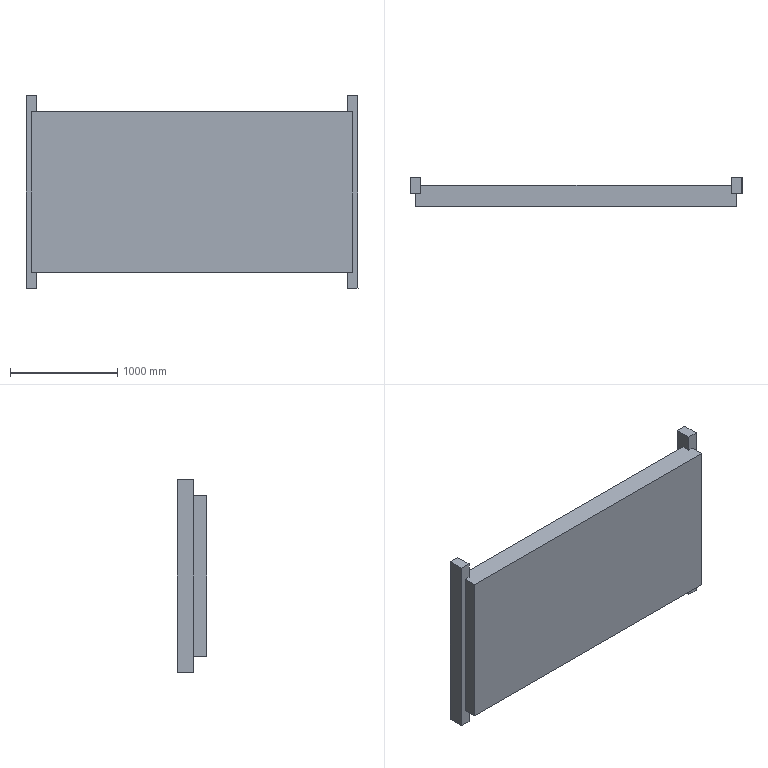Component | SolidWorks | LiftingAndOperatingMechanism-1_21-1 | 1 solid | 18 faces | box 3100 x 275 x 1800 mm | volume 942750000 mm3 | plane 18
build123d program:
from build123d import *

# Parameters (mm, degrees)
SKETCH2_W           = 500
SKETCH2_H           = 800
SKETCH2_W_2         = 440
SKETCH2_H_2         = 740
EXTRUDE_THIN1_DEPTH = 300
SKETCH3_W           = 440
SKETCH3_H           = 240
CUT_EXTRUDE1_DEPTH  = 8353.85
SKETCH4_W           = 740
SKETCH4_H           = 240
CUT_EXTRUDE2_DEPTH  = 8325.662
SKETCH5_W           = 1500
SKETCH5_H           = 3000
BOSS_EXTRUDE1_DEPTH = 100
SKETCH6_W           = 1800
SKETCH6_H           = 150
BOSS_EXTRUDE2_DEPTH = 50
SKETCH9_W           = 1500
SKETCH9_H           = 3000
CUT_EXTRUDE3_DEPTH  = 1944.637


with BuildPart() as part:
    # Sketch2 → Extrude-Thin1 (new body)
    with BuildSketch(Plane(origin=(0, -8000, 0), x_dir=(1, 0, 0), z_dir=(0, 1, 0))):
        with Locations((240, 0)):
            Rectangle(SKETCH2_W, SKETCH2_H)
        with Locations((240, 0)):
            Rectangle(SKETCH2_W_2, SKETCH2_H_2, mode=Mode.SUBTRACT)
    extrude(amount=-EXTRUDE_THIN1_DEPTH)

    # Sketch3 → Cut-Extrude1 (cut, through all)
    with BuildSketch(Plane.XY.offset(400)):
        with Locations((240, -8150)):
            Rectangle(SKETCH3_W, SKETCH3_H)
    extrude(amount=-CUT_EXTRUDE1_DEPTH, mode=Mode.SUBTRACT)

    # Sketch4 → Cut-Extrude2 (cut, through all)
    with BuildSketch(Plane(origin=(490, 0, 0), x_dir=(0, 0, -1), z_dir=(1, 0, 0))):
        with Locations((0, -8150)):
            Rectangle(SKETCH4_W, SKETCH4_H)
    extrude(amount=-CUT_EXTRUDE2_DEPTH, mode=Mode.SUBTRACT)

    # Sketch5 → Boss-Extrude1 (add, symmetric)
    with BuildSketch(Plane.XZ.offset(8300)):
        with Locations((240, 0)):
            Rectangle(SKETCH5_W, SKETCH5_H)
    extrude(amount=BOSS_EXTRUDE1_DEPTH, both=True)

    # Sketch6 → Boss-Extrude2 (add, symmetric)
    with BuildSketch(Plane.XY.offset(1500)):
        with Locations((240, -8400)):
            Rectangle(SKETCH6_W, SKETCH6_H)
    boss_extrude2 = extrude(amount=BOSS_EXTRUDE2_DEPTH, both=True)

    # Mirror1: Boss-Extrude2 across plane
    add(boss_extrude2.mirror(Plane.XY))

    # Sketch9 → Cut-Extrude3 (cut, through all)
    with BuildSketch(Plane(origin=(0, -8200, 0), x_dir=(1, 0, 0), z_dir=(0, 1, 0))):
        with Locations((240, 0)):
            Rectangle(SKETCH9_W, SKETCH9_H)
    extrude(amount=CUT_EXTRUDE3_DEPTH, mode=Mode.SUBTRACT)


solid = part.part

# Placed as in the assembly
solid = solid.moved(Location((-258.963, 11809.183, 6107.842), (180, 90, 0)))
STEP:
#1=COLOUR_RGB('',0.7922,0.8196,0.9333);
#2=FILL_AREA_STYLE_COLOUR('',#1);
#3=FILL_AREA_STYLE('',(#2));
#4=SURFACE_STYLE_FILL_AREA(#3);
#5=SURFACE_SIDE_STYLE('',(#4));
#6=SURFACE_STYLE_USAGE(.BOTH.,#5);
#7=PRESENTATION_STYLE_ASSIGNMENT((#6));
#8=CARTESIAN_POINT('',(46.891,795.637,220.388));
#9=VERTEX_POINT('',#8);
#10=CARTESIAN_POINT('',(-67.282,795.637,220.387));
#11=VERTEX_POINT('',#10);
#12=CARTESIAN_POINT('',(48.86,795.637,220.388));
#13=DIRECTION('',(-1.,-0.,-0.00000094));
#14=VECTOR('',#13,39.37);
#15=LINE('',#12,#14);
#16=EDGE_CURVE('',#9,#11,#15,.T.);
#17=ORIENTED_EDGE('',*,*,#16,.T.);
#18=CARTESIAN_POINT('',(-67.282,795.637,279.443));
#19=VERTEX_POINT('',#18);
#20=CARTESIAN_POINT('',(-67.282,795.637,240.466));
#21=DIRECTION('',(-0.00000094,-0.,1.));
#22=VECTOR('',#21,39.37);
#23=LINE('',#20,#22);
#24=EDGE_CURVE('',#11,#19,#23,.T.);
#25=ORIENTED_EDGE('',*,*,#24,.T.);
#26=CARTESIAN_POINT('',(46.891,795.637,279.443));
#27=VERTEX_POINT('',#26);
#28=CARTESIAN_POINT('',(48.86,795.637,279.443));
#29=DIRECTION('',(1.,0.,0.00000094));
#30=VECTOR('',#29,39.37);
#31=LINE('',#28,#30);
#32=EDGE_CURVE('',#19,#27,#31,.T.);
#33=ORIENTED_EDGE('',*,*,#32,.T.);
#34=CARTESIAN_POINT('',(46.891,795.637,240.466));
#35=DIRECTION('',(0.00000094,0.,-1.));
#36=VECTOR('',#35,39.37);
#37=LINE('',#34,#36);
#38=EDGE_CURVE('',#27,#9,#37,.T.);
#39=ORIENTED_EDGE('',*,*,#38,.T.);
#40=EDGE_LOOP('',(#17,#25,#33,#39));
#41=FACE_OUTER_BOUND('',#40,.T.);
#42=CARTESIAN_POINT('',(-10.195,795.637,240.466));
#43=DIRECTION('',(-0.,1.,0.));
#44=DIRECTION('',(-1.,-0.,-0.00000094));
#45=AXIS2_PLACEMENT_3D('',#42,#43,#44);
#46=PLANE('',#45);
#47=ADVANCED_FACE('',(#41),#46,.T.);
#48=CARTESIAN_POINT('',(-67.282,792.684,279.443));
#49=VERTEX_POINT('',#48);
#50=CARTESIAN_POINT('',(-67.282,795.637,279.443));
#51=DIRECTION('',(-0.,1.,0.));
#52=VECTOR('',#51,39.37);
#53=LINE('',#50,#52);
#54=EDGE_CURVE('',#49,#19,#53,.T.);
#55=ORIENTED_EDGE('',*,*,#54,.F.);
#56=CARTESIAN_POINT('',(-69.251,792.684,279.443));
#57=VERTEX_POINT('',#56);
#58=CARTESIAN_POINT('',(48.86,792.684,279.443));
#59=DIRECTION('',(-1.,-0.,-0.00000094));
#60=VECTOR('',#59,39.37);
#61=LINE('',#58,#60);
#62=EDGE_CURVE('',#49,#57,#61,.T.);
#63=ORIENTED_EDGE('',*,*,#62,.T.);
#64=CARTESIAN_POINT('',(-69.251,787.763,279.443));
#65=VERTEX_POINT('',#64);
#66=CARTESIAN_POINT('',(-69.251,795.637,279.443));
#67=DIRECTION('',(0.,-1.,-0.));
#68=VECTOR('',#67,39.37);
#69=LINE('',#66,#68);
#70=EDGE_CURVE('',#57,#65,#69,.T.);
#71=ORIENTED_EDGE('',*,*,#70,.T.);
#72=CARTESIAN_POINT('',(48.86,787.763,279.443));
#73=VERTEX_POINT('',#72);
#74=CARTESIAN_POINT('',(48.86,787.763,279.443));
#75=DIRECTION('',(1.,0.,0.00000094));
#76=VECTOR('',#75,39.37);
#77=LINE('',#74,#76);
#78=EDGE_CURVE('',#65,#73,#77,.T.);
#79=ORIENTED_EDGE('',*,*,#78,.T.);
#80=CARTESIAN_POINT('',(48.86,792.684,279.443));
#81=VERTEX_POINT('',#80);
#82=CARTESIAN_POINT('',(48.86,795.637,279.443));
#83=DIRECTION('',(0.,-1.,-0.));
#84=VECTOR('',#83,39.37);
#85=LINE('',#82,#84);
#86=EDGE_CURVE('',#81,#73,#85,.T.);
#87=ORIENTED_EDGE('',*,*,#86,.F.);
#88=CARTESIAN_POINT('',(46.891,792.684,279.443));
#89=VERTEX_POINT('',#88);
#90=CARTESIAN_POINT('',(48.86,792.684,279.443));
#91=DIRECTION('',(1.,0.,0.00000094));
#92=VECTOR('',#91,39.37);
#93=LINE('',#90,#92);
#94=EDGE_CURVE('',#89,#81,#93,.T.);
#95=ORIENTED_EDGE('',*,*,#94,.F.);
#96=CARTESIAN_POINT('',(46.891,795.637,279.443));
#97=DIRECTION('',(0.,-1.,-0.));
#98=VECTOR('',#97,39.37);
#99=LINE('',#96,#98);
#100=EDGE_CURVE('',#27,#89,#99,.T.);
#101=ORIENTED_EDGE('',*,*,#100,.F.);
#102=ORIENTED_EDGE('',*,*,#32,.F.);
#103=EDGE_LOOP('',(#55,#63,#71,#79,#87,#95,#101,#102));
#104=FACE_OUTER_BOUND('',#103,.T.);
#105=CARTESIAN_POINT('',(48.86,795.637,279.443));
#106=DIRECTION('',(0.00000094,0.,-1.));
#107=DIRECTION('',(1.,0.,0.00000094));
#108=AXIS2_PLACEMENT_3D('',#105,#106,#107);
#109=PLANE('',#108);
#110=ADVANCED_FACE('',(#104),#109,.F.);
#111=CARTESIAN_POINT('',(48.86,792.684,220.388));
#112=VERTEX_POINT('',#111);
#113=CARTESIAN_POINT('',(48.86,792.684,220.388));
#114=DIRECTION('',(0.00000094,0.,-1.));
#115=VECTOR('',#114,39.37);
#116=LINE('',#113,#115);
#117=EDGE_CURVE('',#81,#112,#116,.T.);
#118=ORIENTED_EDGE('',*,*,#117,.F.);
#119=ORIENTED_EDGE('',*,*,#86,.T.);
#120=CARTESIAN_POINT('',(48.86,787.763,220.388));
#121=VERTEX_POINT('',#120);
#122=CARTESIAN_POINT('',(48.86,787.763,220.388));
#123=DIRECTION('',(0.00000094,0.,-1.));
#124=VECTOR('',#123,39.37);
#125=LINE('',#122,#124);
#126=EDGE_CURVE('',#73,#121,#125,.T.);
#127=ORIENTED_EDGE('',*,*,#126,.T.);
#128=CARTESIAN_POINT('',(48.86,795.637,220.388));
#129=DIRECTION('',(0.,-1.,-0.));
#130=VECTOR('',#129,39.37);
#131=LINE('',#128,#130);
#132=EDGE_CURVE('',#112,#121,#131,.T.);
#133=ORIENTED_EDGE('',*,*,#132,.F.);
#134=EDGE_LOOP('',(#118,#119,#127,#133));
#135=FACE_OUTER_BOUND('',#134,.T.);
#136=CARTESIAN_POINT('',(48.86,795.637,220.388));
#137=DIRECTION('',(-1.,-0.,-0.00000094));
#138=DIRECTION('',(0.00000094,0.,-1.));
#139=AXIS2_PLACEMENT_3D('',#136,#137,#138);
#140=PLANE('',#139);
#141=ADVANCED_FACE('',(#135),#140,.F.);
#142=CARTESIAN_POINT('',(-69.25,792.684,220.387));
#143=VERTEX_POINT('',#142);
#144=CARTESIAN_POINT('',(-69.25,787.763,220.387));
#145=VERTEX_POINT('',#144);
#146=CARTESIAN_POINT('',(-69.25,795.637,220.387));
#147=DIRECTION('',(0.,-1.,-0.));
#148=VECTOR('',#147,39.37);
#149=LINE('',#146,#148);
#150=EDGE_CURVE('',#143,#145,#149,.T.);
#151=ORIENTED_EDGE('',*,*,#150,.F.);
#152=CARTESIAN_POINT('',(-67.282,792.684,220.387));
#153=VERTEX_POINT('',#152);
#154=CARTESIAN_POINT('',(48.86,792.684,220.388));
#155=DIRECTION('',(1.,0.,0.00000094));
#156=VECTOR('',#155,39.37);
#157=LINE('',#154,#156);
#158=EDGE_CURVE('',#143,#153,#157,.T.);
#159=ORIENTED_EDGE('',*,*,#158,.T.);
#160=CARTESIAN_POINT('',(-67.282,795.637,220.387));
#161=DIRECTION('',(0.,-1.,-0.));
#162=VECTOR('',#161,39.37);
#163=LINE('',#160,#162);
#164=EDGE_CURVE('',#11,#153,#163,.T.);
#165=ORIENTED_EDGE('',*,*,#164,.F.);
#166=ORIENTED_EDGE('',*,*,#16,.F.);
#167=CARTESIAN_POINT('',(46.891,792.684,220.388));
#168=VERTEX_POINT('',#167);
#169=CARTESIAN_POINT('',(46.891,795.637,220.388));
#170=DIRECTION('',(-0.,1.,0.));
#171=VECTOR('',#170,39.37);
#172=LINE('',#169,#171);
#173=EDGE_CURVE('',#168,#9,#172,.T.);
#174=ORIENTED_EDGE('',*,*,#173,.F.);
#175=CARTESIAN_POINT('',(48.86,792.684,220.388));
#176=DIRECTION('',(-1.,-0.,-0.00000094));
#177=VECTOR('',#176,39.37);
#178=LINE('',#175,#177);
#179=EDGE_CURVE('',#112,#168,#178,.T.);
#180=ORIENTED_EDGE('',*,*,#179,.F.);
#181=ORIENTED_EDGE('',*,*,#132,.T.);
#182=CARTESIAN_POINT('',(48.86,787.763,220.388));
#183=DIRECTION('',(-1.,-0.,-0.00000094));
#184=VECTOR('',#183,39.37);
#185=LINE('',#182,#184);
#186=EDGE_CURVE('',#121,#145,#185,.T.);
#187=ORIENTED_EDGE('',*,*,#186,.T.);
#188=EDGE_LOOP('',(#151,#159,#165,#166,#174,#180,#181,#187));
#189=FACE_OUTER_BOUND('',#188,.T.);
#190=CARTESIAN_POINT('',(48.86,795.637,220.388));
#191=DIRECTION('',(-0.00000094,-0.,1.));
#192=DIRECTION('',(-1.,-0.,-0.00000094));
#193=AXIS2_PLACEMENT_3D('',#190,#191,#192);
#194=PLANE('',#193);
#195=ADVANCED_FACE('',(#189),#194,.F.);
#196=ORIENTED_EDGE('',*,*,#78,.F.);
#197=CARTESIAN_POINT('',(-69.25,787.763,220.387));
#198=DIRECTION('',(-0.00000094,-0.,1.));
#199=VECTOR('',#198,39.37);
#200=LINE('',#197,#199);
#201=EDGE_CURVE('',#145,#65,#200,.T.);
#202=ORIENTED_EDGE('',*,*,#201,.F.);
#203=ORIENTED_EDGE('',*,*,#186,.F.);
#204=ORIENTED_EDGE('',*,*,#126,.F.);
#205=EDGE_LOOP('',(#196,#202,#203,#204));
#206=FACE_OUTER_BOUND('',#205,.T.);
#207=CARTESIAN_POINT('',(-10.195,787.763,240.466));
#208=DIRECTION('',(-0.,1.,0.));
#209=DIRECTION('',(-1.,-0.,-0.00000094));
#210=AXIS2_PLACEMENT_3D('',#207,#208,#209);
#211=PLANE('',#210);
#212=ADVANCED_FACE('',(#206),#211,.F.);
#213=ORIENTED_EDGE('',*,*,#70,.F.);
#214=CARTESIAN_POINT('',(-69.25,792.684,220.387));
#215=DIRECTION('',(0.00000094,0.,-1.));
#216=VECTOR('',#215,39.37);
#217=LINE('',#214,#216);
#218=EDGE_CURVE('',#57,#143,#217,.T.);
#219=ORIENTED_EDGE('',*,*,#218,.T.);
#220=ORIENTED_EDGE('',*,*,#150,.T.);
#221=ORIENTED_EDGE('',*,*,#201,.T.);
#222=EDGE_LOOP('',(#213,#219,#220,#221));
#223=FACE_OUTER_BOUND('',#222,.T.);
#224=CARTESIAN_POINT('',(-69.25,795.637,220.387));
#225=DIRECTION('',(1.,0.,0.00000094));
#226=DIRECTION('',(-0.00000094,-0.,1.));
#227=AXIS2_PLACEMENT_3D('',#224,#225,#226);
#228=PLANE('',#227);
#229=ADVANCED_FACE('',(#223),#228,.F.);
#230=CARTESIAN_POINT('',(46.891,792.684,285.348));
#231=VERTEX_POINT('',#230);
#232=CARTESIAN_POINT('',(46.891,792.684,214.482));
#233=DIRECTION('',(0.00000094,0.,-1.));
#234=VECTOR('',#233,39.37);
#235=LINE('',#232,#234);
#236=EDGE_CURVE('',#231,#89,#235,.T.);
#237=ORIENTED_EDGE('',*,*,#236,.T.);
#238=ORIENTED_EDGE('',*,*,#94,.T.);
#239=ORIENTED_EDGE('',*,*,#117,.T.);
#240=ORIENTED_EDGE('',*,*,#179,.T.);
#241=CARTESIAN_POINT('',(46.891,792.684,214.482));
#242=VERTEX_POINT('',#241);
#243=CARTESIAN_POINT('',(46.891,792.684,214.482));
#244=DIRECTION('',(0.00000094,0.,-1.));
#245=VECTOR('',#244,39.37);
#246=LINE('',#243,#245);
#247=EDGE_CURVE('',#168,#242,#246,.T.);
#248=ORIENTED_EDGE('',*,*,#247,.T.);
#249=CARTESIAN_POINT('',(50.828,792.684,214.482));
#250=VERTEX_POINT('',#249);
#251=CARTESIAN_POINT('',(50.828,792.684,214.482));
#252=DIRECTION('',(-1.,-0.,-0.00000094));
#253=VECTOR('',#252,39.37);
#254=LINE('',#251,#253);
#255=EDGE_CURVE('',#250,#242,#254,.T.);
#256=ORIENTED_EDGE('',*,*,#255,.F.);
#257=CARTESIAN_POINT('',(50.828,792.684,285.348));
#258=VERTEX_POINT('',#257);
#259=CARTESIAN_POINT('',(50.828,792.684,214.482));
#260=DIRECTION('',(0.00000094,0.,-1.));
#261=VECTOR('',#260,39.37);
#262=LINE('',#259,#261);
#263=EDGE_CURVE('',#258,#250,#262,.T.);
#264=ORIENTED_EDGE('',*,*,#263,.F.);
#265=CARTESIAN_POINT('',(50.828,792.684,285.348));
#266=DIRECTION('',(-1.,-0.,-0.00000094));
#267=VECTOR('',#266,39.37);
#268=LINE('',#265,#267);
#269=EDGE_CURVE('',#258,#231,#268,.T.);
#270=ORIENTED_EDGE('',*,*,#269,.T.);
#271=EDGE_LOOP('',(#237,#238,#239,#240,#248,#256,#264,#270));
#272=FACE_OUTER_BOUND('',#271,.T.);
#273=CARTESIAN_POINT('',(50.828,792.684,214.482));
#274=DIRECTION('',(-0.,1.,0.));
#275=DIRECTION('',(-1.,-0.,-0.00000094));
#276=AXIS2_PLACEMENT_3D('',#273,#274,#275);
#277=PLANE('',#276);
#278=ADVANCED_FACE('',(#272),#277,.F.);
#279=ORIENTED_EDGE('',*,*,#38,.F.);
#280=ORIENTED_EDGE('',*,*,#100,.T.);
#281=ORIENTED_EDGE('',*,*,#236,.F.);
#282=CARTESIAN_POINT('',(46.891,798.59,285.348));
#283=VERTEX_POINT('',#282);
#284=CARTESIAN_POINT('',(46.891,792.684,285.348));
#285=DIRECTION('',(0.,-1.,-0.));
#286=VECTOR('',#285,39.37);
#287=LINE('',#284,#286);
#288=EDGE_CURVE('',#283,#231,#287,.T.);
#289=ORIENTED_EDGE('',*,*,#288,.F.);
#290=CARTESIAN_POINT('',(46.891,798.59,214.482));
#291=VERTEX_POINT('',#290);
#292=CARTESIAN_POINT('',(46.891,798.59,214.482));
#293=DIRECTION('',(-0.00000094,-0.,1.));
#294=VECTOR('',#293,39.37);
#295=LINE('',#292,#294);
#296=EDGE_CURVE('',#291,#283,#295,.T.);
#297=ORIENTED_EDGE('',*,*,#296,.F.);
#298=CARTESIAN_POINT('',(46.891,792.684,214.482));
#299=DIRECTION('',(-0.,1.,0.));
#300=VECTOR('',#299,39.37);
#301=LINE('',#298,#300);
#302=EDGE_CURVE('',#242,#291,#301,.T.);
#303=ORIENTED_EDGE('',*,*,#302,.F.);
#304=ORIENTED_EDGE('',*,*,#247,.F.);
#305=ORIENTED_EDGE('',*,*,#173,.T.);
#306=EDGE_LOOP('',(#279,#280,#281,#289,#297,#303,#304,#305));
#307=FACE_OUTER_BOUND('',#306,.T.);
#308=CARTESIAN_POINT('',(46.891,464.928,240.466));
#309=DIRECTION('',(1.,0.,0.00000094));
#310=DIRECTION('',(-0.00000094,-0.,1.));
#311=AXIS2_PLACEMENT_3D('',#308,#309,#310);
#312=PLANE('',#311);
#313=ADVANCED_FACE('',(#307),#312,.F.);
#314=ORIENTED_EDGE('',*,*,#288,.T.);
#315=ORIENTED_EDGE('',*,*,#269,.F.);
#316=CARTESIAN_POINT('',(50.828,798.59,285.348));
#317=VERTEX_POINT('',#316);
#318=CARTESIAN_POINT('',(50.828,792.684,285.348));
#319=DIRECTION('',(0.,-1.,-0.));
#320=VECTOR('',#319,39.37);
#321=LINE('',#318,#320);
#322=EDGE_CURVE('',#317,#258,#321,.T.);
#323=ORIENTED_EDGE('',*,*,#322,.F.);
#324=CARTESIAN_POINT('',(50.828,798.59,285.348));
#325=DIRECTION('',(-1.,-0.,-0.00000094));
#326=VECTOR('',#325,39.37);
#327=LINE('',#324,#326);
#328=EDGE_CURVE('',#317,#283,#327,.T.);
#329=ORIENTED_EDGE('',*,*,#328,.T.);
#330=EDGE_LOOP('',(#314,#315,#323,#329));
#331=FACE_OUTER_BOUND('',#330,.T.);
#332=CARTESIAN_POINT('',(50.828,792.684,285.348));
#333=DIRECTION('',(0.00000094,0.,-1.));
#334=DIRECTION('',(1.,0.,0.00000094));
#335=AXIS2_PLACEMENT_3D('',#332,#333,#334);
#336=PLANE('',#335);
#337=ADVANCED_FACE('',(#331),#336,.F.);
#338=ORIENTED_EDGE('',*,*,#302,.T.);
#339=CARTESIAN_POINT('',(50.828,798.59,214.482));
#340=VERTEX_POINT('',#339);
#341=CARTESIAN_POINT('',(50.828,798.59,214.482));
#342=DIRECTION('',(-1.,-0.,-0.00000094));
#343=VECTOR('',#342,39.37);
#344=LINE('',#341,#343);
#345=EDGE_CURVE('',#340,#291,#344,.T.);
#346=ORIENTED_EDGE('',*,*,#345,.F.);
#347=CARTESIAN_POINT('',(50.828,792.684,214.482));
#348=DIRECTION('',(-0.,1.,0.));
#349=VECTOR('',#348,39.37);
#350=LINE('',#347,#349);
#351=EDGE_CURVE('',#250,#340,#350,.T.);
#352=ORIENTED_EDGE('',*,*,#351,.F.);
#353=ORIENTED_EDGE('',*,*,#255,.T.);
#354=EDGE_LOOP('',(#338,#346,#352,#353));
#355=FACE_OUTER_BOUND('',#354,.T.);
#356=CARTESIAN_POINT('',(50.828,792.684,214.482));
#357=DIRECTION('',(-0.00000094,-0.,1.));
#358=DIRECTION('',(-1.,-0.,-0.00000094));
#359=AXIS2_PLACEMENT_3D('',#356,#357,#358);
#360=PLANE('',#359);
#361=ADVANCED_FACE('',(#355),#360,.F.);
#362=ORIENTED_EDGE('',*,*,#296,.T.);
#363=ORIENTED_EDGE('',*,*,#328,.F.);
#364=CARTESIAN_POINT('',(50.828,798.59,214.482));
#365=DIRECTION('',(-0.00000094,-0.,1.));
#366=VECTOR('',#365,39.37);
#367=LINE('',#364,#366);
#368=EDGE_CURVE('',#340,#317,#367,.T.);
#369=ORIENTED_EDGE('',*,*,#368,.F.);
#370=ORIENTED_EDGE('',*,*,#345,.T.);
#371=EDGE_LOOP('',(#362,#363,#369,#370));
#372=FACE_OUTER_BOUND('',#371,.T.);
#373=CARTESIAN_POINT('',(50.828,798.59,214.482));
#374=DIRECTION('',(0.,-1.,-0.));
#375=DIRECTION('',(1.,0.,0.00000094));
#376=AXIS2_PLACEMENT_3D('',#373,#374,#375);
#377=PLANE('',#376);
#378=ADVANCED_FACE('',(#372),#377,.F.);
#379=ORIENTED_EDGE('',*,*,#322,.T.);
#380=ORIENTED_EDGE('',*,*,#263,.T.);
#381=ORIENTED_EDGE('',*,*,#351,.T.);
#382=ORIENTED_EDGE('',*,*,#368,.T.);
#383=EDGE_LOOP('',(#379,#380,#381,#382));
#384=FACE_OUTER_BOUND('',#383,.T.);
#385=CARTESIAN_POINT('',(50.828,464.928,240.466));
#386=DIRECTION('',(1.,0.,0.00000094));
#387=DIRECTION('',(-0.00000094,-0.,1.));
#388=AXIS2_PLACEMENT_3D('',#385,#386,#387);
#389=PLANE('',#388);
#390=ADVANCED_FACE('',(#384),#389,.T.);
#391=CARTESIAN_POINT('',(-67.282,792.684,285.348));
#392=VERTEX_POINT('',#391);
#393=CARTESIAN_POINT('',(-67.282,792.684,214.482));
#394=DIRECTION('',(0.00000094,0.,-1.));
#395=VECTOR('',#394,39.37);
#396=LINE('',#393,#395);
#397=EDGE_CURVE('',#392,#49,#396,.T.);
#398=ORIENTED_EDGE('',*,*,#397,.T.);
#399=ORIENTED_EDGE('',*,*,#54,.T.);
#400=ORIENTED_EDGE('',*,*,#24,.F.);
#401=ORIENTED_EDGE('',*,*,#164,.T.);
#402=CARTESIAN_POINT('',(-67.282,792.684,214.482));
#403=VERTEX_POINT('',#402);
#404=CARTESIAN_POINT('',(-67.282,792.684,214.482));
#405=DIRECTION('',(0.00000094,0.,-1.));
#406=VECTOR('',#405,39.37);
#407=LINE('',#404,#406);
#408=EDGE_CURVE('',#153,#403,#407,.T.);
#409=ORIENTED_EDGE('',*,*,#408,.T.);
#410=CARTESIAN_POINT('',(-67.282,798.59,214.482));
#411=VERTEX_POINT('',#410);
#412=CARTESIAN_POINT('',(-67.282,792.684,214.482));
#413=DIRECTION('',(-0.,1.,0.));
#414=VECTOR('',#413,39.37);
#415=LINE('',#412,#414);
#416=EDGE_CURVE('',#403,#411,#415,.T.);
#417=ORIENTED_EDGE('',*,*,#416,.T.);
#418=CARTESIAN_POINT('',(-67.282,798.59,285.348));
#419=VERTEX_POINT('',#418);
#420=CARTESIAN_POINT('',(-67.282,798.59,214.482));
#421=DIRECTION('',(-0.00000094,-0.,1.));
#422=VECTOR('',#421,39.37);
#423=LINE('',#420,#422);
#424=EDGE_CURVE('',#411,#419,#423,.T.);
#425=ORIENTED_EDGE('',*,*,#424,.T.);
#426=CARTESIAN_POINT('',(-67.282,792.684,285.348));
#427=DIRECTION('',(0.,-1.,-0.));
#428=VECTOR('',#427,39.37);
#429=LINE('',#426,#428);
#430=EDGE_CURVE('',#419,#392,#429,.T.);
#431=ORIENTED_EDGE('',*,*,#430,.T.);
#432=EDGE_LOOP('',(#398,#399,#400,#401,#409,#417,#425,#431));
#433=FACE_OUTER_BOUND('',#432,.T.);
#434=CARTESIAN_POINT('',(-67.282,464.928,240.466));
#435=DIRECTION('',(-1.,-0.,-0.00000094));
#436=DIRECTION('',(-0.00000094,-0.,1.));
#437=AXIS2_PLACEMENT_3D('',#434,#435,#436);
#438=PLANE('',#437);
#439=ADVANCED_FACE('',(#433),#438,.F.);
#440=ORIENTED_EDGE('',*,*,#62,.F.);
#441=ORIENTED_EDGE('',*,*,#397,.F.);
#442=CARTESIAN_POINT('',(-71.219,792.684,285.348));
#443=VERTEX_POINT('',#442);
#444=CARTESIAN_POINT('',(-71.219,792.684,285.348));
#445=DIRECTION('',(1.,0.,0.00000094));
#446=VECTOR('',#445,39.37);
#447=LINE('',#444,#446);
#448=EDGE_CURVE('',#443,#392,#447,.T.);
#449=ORIENTED_EDGE('',*,*,#448,.F.);
#450=CARTESIAN_POINT('',(-71.219,792.684,214.482));
#451=VERTEX_POINT('',#450);
#452=CARTESIAN_POINT('',(-71.219,792.684,214.482));
#453=DIRECTION('',(0.00000094,0.,-1.));
#454=VECTOR('',#453,39.37);
#455=LINE('',#452,#454);
#456=EDGE_CURVE('',#443,#451,#455,.T.);
#457=ORIENTED_EDGE('',*,*,#456,.T.);
#458=CARTESIAN_POINT('',(-71.219,792.684,214.482));
#459=DIRECTION('',(1.,0.,0.00000094));
#460=VECTOR('',#459,39.37);
#461=LINE('',#458,#460);
#462=EDGE_CURVE('',#451,#403,#461,.T.);
#463=ORIENTED_EDGE('',*,*,#462,.T.);
#464=ORIENTED_EDGE('',*,*,#408,.F.);
#465=ORIENTED_EDGE('',*,*,#158,.F.);
#466=ORIENTED_EDGE('',*,*,#218,.F.);
#467=EDGE_LOOP('',(#440,#441,#449,#457,#463,#464,#465,#466));
#468=FACE_OUTER_BOUND('',#467,.T.);
#469=CARTESIAN_POINT('',(-71.219,792.684,214.482));
#470=DIRECTION('',(0.,-1.,-0.));
#471=DIRECTION('',(1.,0.,0.00000094));
#472=AXIS2_PLACEMENT_3D('',#469,#470,#471);
#473=PLANE('',#472);
#474=ADVANCED_FACE('',(#468),#473,.T.);
#475=ORIENTED_EDGE('',*,*,#430,.F.);
#476=CARTESIAN_POINT('',(-71.219,798.59,285.348));
#477=VERTEX_POINT('',#476);
#478=CARTESIAN_POINT('',(-71.219,798.59,285.348));
#479=DIRECTION('',(1.,0.,0.00000094));
#480=VECTOR('',#479,39.37);
#481=LINE('',#478,#480);
#482=EDGE_CURVE('',#477,#419,#481,.T.);
#483=ORIENTED_EDGE('',*,*,#482,.F.);
#484=CARTESIAN_POINT('',(-71.219,792.684,285.348));
#485=DIRECTION('',(0.,-1.,-0.));
#486=VECTOR('',#485,39.37);
#487=LINE('',#484,#486);
#488=EDGE_CURVE('',#477,#443,#487,.T.);
#489=ORIENTED_EDGE('',*,*,#488,.T.);
#490=ORIENTED_EDGE('',*,*,#448,.T.);
#491=EDGE_LOOP('',(#475,#483,#489,#490));
#492=FACE_OUTER_BOUND('',#491,.T.);
#493=CARTESIAN_POINT('',(-71.219,792.684,285.348));
#494=DIRECTION('',(-0.00000094,-0.,1.));
#495=DIRECTION('',(-1.,-0.,-0.00000094));
#496=AXIS2_PLACEMENT_3D('',#493,#494,#495);
#497=PLANE('',#496);
#498=ADVANCED_FACE('',(#492),#497,.T.);
#499=ORIENTED_EDGE('',*,*,#424,.F.);
#500=CARTESIAN_POINT('',(-71.219,798.59,214.482));
#501=VERTEX_POINT('',#500);
#502=CARTESIAN_POINT('',(-71.219,798.59,214.482));
#503=DIRECTION('',(1.,0.,0.00000094));
#504=VECTOR('',#503,39.37);
#505=LINE('',#502,#504);
#506=EDGE_CURVE('',#501,#411,#505,.T.);
#507=ORIENTED_EDGE('',*,*,#506,.F.);
#508=CARTESIAN_POINT('',(-71.219,798.59,214.482));
#509=DIRECTION('',(-0.00000094,-0.,1.));
#510=VECTOR('',#509,39.37);
#511=LINE('',#508,#510);
#512=EDGE_CURVE('',#501,#477,#511,.T.);
#513=ORIENTED_EDGE('',*,*,#512,.T.);
#514=ORIENTED_EDGE('',*,*,#482,.T.);
#515=EDGE_LOOP('',(#499,#507,#513,#514));
#516=FACE_OUTER_BOUND('',#515,.T.);
#517=CARTESIAN_POINT('',(-71.219,798.59,214.482));
#518=DIRECTION('',(-0.,1.,0.));
#519=DIRECTION('',(-1.,-0.,-0.00000094));
#520=AXIS2_PLACEMENT_3D('',#517,#518,#519);
#521=PLANE('',#520);
#522=ADVANCED_FACE('',(#516),#521,.T.);
#523=ORIENTED_EDGE('',*,*,#416,.F.);
#524=ORIENTED_EDGE('',*,*,#462,.F.);
#525=CARTESIAN_POINT('',(-71.219,792.684,214.482));
#526=DIRECTION('',(-0.,1.,0.));
#527=VECTOR('',#526,39.37);
#528=LINE('',#525,#527);
#529=EDGE_CURVE('',#451,#501,#528,.T.);
#530=ORIENTED_EDGE('',*,*,#529,.T.);
#531=ORIENTED_EDGE('',*,*,#506,.T.);
#532=EDGE_LOOP('',(#523,#524,#530,#531));
#533=FACE_OUTER_BOUND('',#532,.T.);
#534=CARTESIAN_POINT('',(-71.219,792.684,214.482));
#535=DIRECTION('',(0.00000094,0.,-1.));
#536=DIRECTION('',(1.,0.,0.00000094));
#537=AXIS2_PLACEMENT_3D('',#534,#535,#536);
#538=PLANE('',#537);
#539=ADVANCED_FACE('',(#533),#538,.T.);
#540=ORIENTED_EDGE('',*,*,#488,.F.);
#541=ORIENTED_EDGE('',*,*,#512,.F.);
#542=ORIENTED_EDGE('',*,*,#529,.F.);
#543=ORIENTED_EDGE('',*,*,#456,.F.);
#544=EDGE_LOOP('',(#540,#541,#542,#543));
#545=FACE_OUTER_BOUND('',#544,.T.);
#546=CARTESIAN_POINT('',(-71.219,464.928,240.466));
#547=DIRECTION('',(-1.,-0.,-0.00000094));
#548=DIRECTION('',(-0.00000094,-0.,1.));
#549=AXIS2_PLACEMENT_3D('',#546,#547,#548);
#550=PLANE('',#549);
#551=ADVANCED_FACE('',(#545),#550,.T.);
#552=CLOSED_SHELL('',(#47,#110,#141,#195,#212,#229,#278,#313,#337,#361,#378,#390,#439,#474,#498,#522,#539,#551));
#553=MANIFOLD_SOLID_BREP('',#552);
#554=STYLED_ITEM('',(#7),#553);
#555=(LENGTH_UNIT()NAMED_UNIT(*)SI_UNIT($,.METRE.));
#556=LENGTH_MEASURE_WITH_UNIT(LENGTH_MEASURE(0.0254),#555);
#557=DIMENSIONAL_EXPONENTS(1.,0.,0.,0.,0.,0.,0.);
#558=(CONVERSION_BASED_UNIT('',#556)LENGTH_UNIT()NAMED_UNIT(#557));
#559=UNCERTAINTY_MEASURE_WITH_UNIT(LENGTH_MEASURE(0.00001),#558,'','');
#560=(NAMED_UNIT(*)PLANE_ANGLE_UNIT()SI_UNIT($,.RADIAN.));
#561=(NAMED_UNIT(*)SI_UNIT($,.STERADIAN.)SOLID_ANGLE_UNIT());
#562=(GEOMETRIC_REPRESENTATION_CONTEXT(3)GLOBAL_UNCERTAINTY_ASSIGNED_CONTEXT((#559))GLOBAL_UNIT_ASSIGNED_CONTEXT((#558,#560,#561))REPRESENTATION_CONTEXT('',''));
#563=MECHANICAL_DESIGN_GEOMETRIC_PRESENTATION_REPRESENTATION('',(#554),#562);
#564=CARTESIAN_POINT('',(0.,0.,0.));
#565=DIRECTION('',(0.,0.,1.));
#566=DIRECTION('',(1.,0.,0.));
#567=AXIS2_PLACEMENT_3D('',#564,#565,#566);
#568=(LENGTH_UNIT()NAMED_UNIT(*)SI_UNIT($,.METRE.));
#569=LENGTH_MEASURE_WITH_UNIT(LENGTH_MEASURE(0.0254),#568);
#570=DIMENSIONAL_EXPONENTS(1.,0.,0.,0.,0.,0.,0.);
#571=(CONVERSION_BASED_UNIT('',#569)LENGTH_UNIT()NAMED_UNIT(#570));
#572=UNCERTAINTY_MEASURE_WITH_UNIT(LENGTH_MEASURE(0.00001),#571,'','');
#573=(NAMED_UNIT(*)PLANE_ANGLE_UNIT()SI_UNIT($,.RADIAN.));
#574=(NAMED_UNIT(*)SI_UNIT($,.STERADIAN.)SOLID_ANGLE_UNIT());
#575=(GEOMETRIC_REPRESENTATION_CONTEXT(3)GLOBAL_UNCERTAINTY_ASSIGNED_CONTEXT((#572))GLOBAL_UNIT_ASSIGNED_CONTEXT((#571,#573,#574))REPRESENTATION_CONTEXT('',''));
#576=ADVANCED_BREP_SHAPE_REPRESENTATION('',(#553,#567),#575);
#577=PRESENTATION_LAYER_ASSIGNMENT('','',(#554));